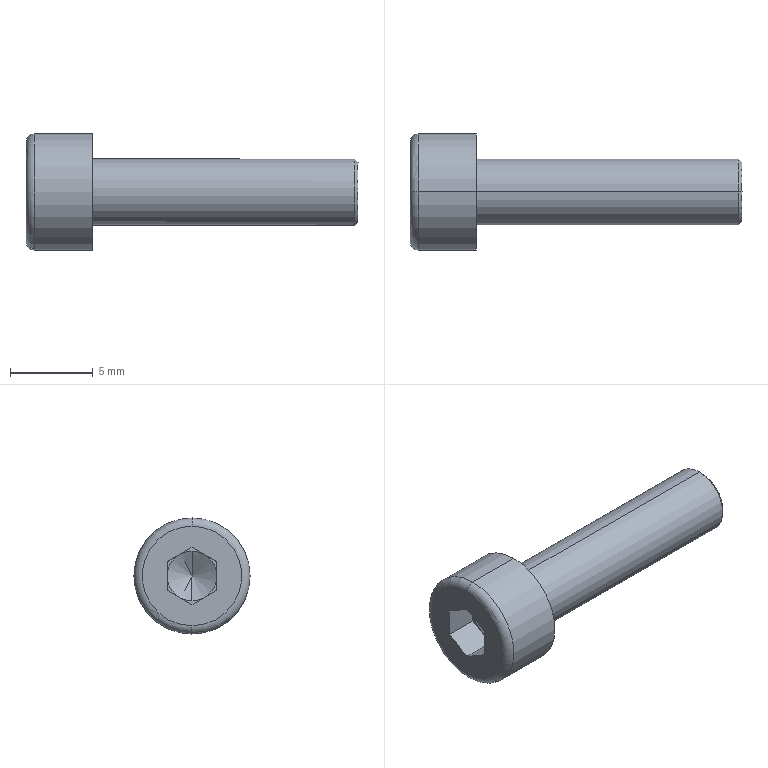Component | SolidWorks | hexagon socket head cap screws gb-34 | 1 solid | 25 faces | box 20.01 x 7 x 7 mm | volume 336 mm3 | plane 15 | cone 4 | cylinder 4 | torus 2 | commonest cylinder face diameters 4 x2 7 x2
STEP:
#1=CARTESIAN_POINT('',(-1.336,35.871,32.265));
#2=VERTEX_POINT('',#1);
#3=CARTESIAN_POINT('',(-1.336,35.871,32.407));
#4=VERTEX_POINT('',#3);
#5=CARTESIAN_POINT('',(-1.336,35.871,32.336));
#6=DIRECTION('',(1.,0.,-0.00108));
#7=DIRECTION('',(-0.00108,0.,-1.));
#8=AXIS2_PLACEMENT_3D('',#5,#6,#7);
#9=CIRCLE('',#8,0.07087);
#10=EDGE_CURVE('',#2,#4,#9,.T.);
#11=ORIENTED_EDGE('',*,*,#10,.F.);
#12=CARTESIAN_POINT('',(-1.344,35.871,32.257));
#13=VERTEX_POINT('',#12);
#14=CARTESIAN_POINT('',(-1.336,35.871,32.265));
#15=DIRECTION('',(-0.7079,0.,-0.7063));
#16=VECTOR('',#15,39.37);
#17=LINE('',#14,#16);
#18=EDGE_CURVE('',#2,#13,#17,.T.);
#19=ORIENTED_EDGE('',*,*,#18,.T.);
#20=CARTESIAN_POINT('',(-1.344,35.871,32.415));
#21=VERTEX_POINT('',#20);
#22=CARTESIAN_POINT('',(-1.344,35.871,32.336));
#23=DIRECTION('',(-1.,-0.,0.00108));
#24=DIRECTION('',(-0.00108,0.,-1.));
#25=AXIS2_PLACEMENT_3D('',#22,#23,#24);
#26=CIRCLE('',#25,0.07874);
#27=EDGE_CURVE('',#21,#13,#26,.T.);
#28=ORIENTED_EDGE('',*,*,#27,.F.);
#29=CARTESIAN_POINT('',(-1.336,35.871,32.407));
#30=DIRECTION('',(-0.7063,-0.,0.7079));
#31=VECTOR('',#30,39.37);
#32=LINE('',#29,#31);
#33=EDGE_CURVE('',#4,#21,#32,.T.);
#34=ORIENTED_EDGE('',*,*,#33,.F.);
#35=EDGE_LOOP('',(#11,#19,#28,#34));
#36=FACE_OUTER_BOUND('',#35,.T.);
#37=CARTESIAN_POINT('',(-1.336,35.871,32.336));
#38=DIRECTION('',(-1.,-0.,0.00108));
#39=DIRECTION('',(0.00108,-0.,1.));
#40=AXIS2_PLACEMENT_3D('',#37,#38,#39);
#41=CONICAL_SURFACE('',#40,0.07087,0.7854);
#42=ADVANCED_FACE('',(#36),#41,.T.);
#43=CARTESIAN_POINT('',(-2.123,35.871,32.455));
#44=VERTEX_POINT('',#43);
#45=CARTESIAN_POINT('',(-2.124,35.871,32.219));
#46=VERTEX_POINT('',#45);
#47=CARTESIAN_POINT('',(-2.123,35.871,32.337));
#48=DIRECTION('',(-1.,-0.,0.00108));
#49=DIRECTION('',(-0.00108,0.,-1.));
#50=AXIS2_PLACEMENT_3D('',#47,#48,#49);
#51=CIRCLE('',#50,0.1181);
#52=EDGE_CURVE('',#44,#46,#51,.T.);
#53=ORIENTED_EDGE('',*,*,#52,.F.);
#54=CARTESIAN_POINT('',(-2.104,35.871,32.475));
#55=VERTEX_POINT('',#54);
#56=CARTESIAN_POINT('',(-2.104,35.871,32.455));
#57=DIRECTION('',(0.,1.,0.));
#58=DIRECTION('',(0.,-0.,1.));
#59=AXIS2_PLACEMENT_3D('',#56,#57,#58);
#60=CIRCLE('',#59,0.01969);
#61=EDGE_CURVE('',#44,#55,#60,.T.);
#62=ORIENTED_EDGE('',*,*,#61,.T.);
#63=CARTESIAN_POINT('',(-2.104,35.871,32.199));
#64=VERTEX_POINT('',#63);
#65=CARTESIAN_POINT('',(-2.104,35.871,32.337));
#66=DIRECTION('',(1.,0.,-0.00108));
#67=DIRECTION('',(-0.00108,0.,-1.));
#68=AXIS2_PLACEMENT_3D('',#65,#66,#67);
#69=CIRCLE('',#68,0.1378);
#70=EDGE_CURVE('',#64,#55,#69,.T.);
#71=ORIENTED_EDGE('',*,*,#70,.F.);
#72=CARTESIAN_POINT('',(-2.104,35.871,32.219));
#73=DIRECTION('',(-0.,-1.,-0.));
#74=DIRECTION('',(0.,0.,-1.));
#75=AXIS2_PLACEMENT_3D('',#72,#73,#74);
#76=CIRCLE('',#75,0.01969);
#77=EDGE_CURVE('',#46,#64,#76,.T.);
#78=ORIENTED_EDGE('',*,*,#77,.F.);
#79=EDGE_LOOP('',(#53,#62,#71,#78));
#80=FACE_OUTER_BOUND('',#79,.T.);
#81=CARTESIAN_POINT('',(-2.104,35.871,32.337));
#82=DIRECTION('',(1.,0.,-0.00108));
#83=DIRECTION('',(-0.00108,0.,-1.));
#84=AXIS2_PLACEMENT_3D('',#81,#82,#83);
#85=TOROIDAL_SURFACE('',#84,0.1181,0.01969);
#86=ADVANCED_FACE('',(#80),#85,.T.);
#87=CARTESIAN_POINT('',(-2.011,35.871,32.337));
#88=VERTEX_POINT('',#87);
#89=CARTESIAN_POINT('',(-2.045,35.871,32.396));
#90=VERTEX_POINT('',#89);
#91=CARTESIAN_POINT('',(-2.045,35.871,32.396));
#92=DIRECTION('',(-0.4991,-0.,0.8666));
#93=VECTOR('',#92,39.37);
#94=LINE('',#91,#93);
#95=EDGE_CURVE('',#88,#90,#94,.T.);
#96=ORIENTED_EDGE('',*,*,#95,.F.);
#97=CARTESIAN_POINT('',(-2.045,35.871,32.278));
#98=VERTEX_POINT('',#97);
#99=CARTESIAN_POINT('',(-2.045,35.871,32.278));
#100=DIRECTION('',(-0.5009,0.,-0.8655));
#101=VECTOR('',#100,39.37);
#102=LINE('',#99,#101);
#103=EDGE_CURVE('',#88,#98,#102,.T.);
#104=ORIENTED_EDGE('',*,*,#103,.T.);
#105=CARTESIAN_POINT('',(-2.045,35.841,32.286));
#106=VERTEX_POINT('',#105);
#107=CARTESIAN_POINT('',(-2.045,35.871,32.337));
#108=DIRECTION('',(1.,0.,-0.00108));
#109=DIRECTION('',(0.00108,-0.,1.));
#110=AXIS2_PLACEMENT_3D('',#107,#108,#109);
#111=CIRCLE('',#110,0.05906);
#112=EDGE_CURVE('',#106,#98,#111,.T.);
#113=ORIENTED_EDGE('',*,*,#112,.F.);
#114=CARTESIAN_POINT('',(-2.045,35.811,32.337));
#115=VERTEX_POINT('',#114);
#116=CARTESIAN_POINT('',(-2.045,35.871,32.337));
#117=DIRECTION('',(1.,0.,-0.00108));
#118=DIRECTION('',(0.00108,-0.,1.));
#119=AXIS2_PLACEMENT_3D('',#116,#117,#118);
#120=CIRCLE('',#119,0.05906);
#121=EDGE_CURVE('',#115,#106,#120,.T.);
#122=ORIENTED_EDGE('',*,*,#121,.F.);
#123=CARTESIAN_POINT('',(-2.045,35.841,32.388));
#124=VERTEX_POINT('',#123);
#125=CARTESIAN_POINT('',(-2.045,35.871,32.337));
#126=DIRECTION('',(1.,0.,-0.00108));
#127=DIRECTION('',(0.00108,-0.,1.));
#128=AXIS2_PLACEMENT_3D('',#125,#126,#127);
#129=CIRCLE('',#128,0.05906);
#130=EDGE_CURVE('',#124,#115,#129,.T.);
#131=ORIENTED_EDGE('',*,*,#130,.F.);
#132=CARTESIAN_POINT('',(-2.045,35.871,32.337));
#133=DIRECTION('',(1.,0.,-0.00108));
#134=DIRECTION('',(0.00108,-0.,1.));
#135=AXIS2_PLACEMENT_3D('',#132,#133,#134);
#136=CIRCLE('',#135,0.05906);
#137=EDGE_CURVE('',#90,#124,#136,.T.);
#138=ORIENTED_EDGE('',*,*,#137,.F.);
#139=EDGE_LOOP('',(#96,#104,#113,#122,#131,#138));
#140=FACE_OUTER_BOUND('',#139,.T.);
#141=CARTESIAN_POINT('',(-2.045,35.871,32.337));
#142=DIRECTION('',(-1.,-0.,0.00108));
#143=DIRECTION('',(0.00108,-0.,1.));
#144=AXIS2_PLACEMENT_3D('',#141,#142,#143);
#145=CONICAL_SURFACE('',#144,0.05906,1.047);
#146=ADVANCED_FACE('',(#140),#145,.F.);
#147=ORIENTED_EDGE('',*,*,#27,.T.);
#148=CARTESIAN_POINT('',(-1.966,35.871,32.258));
#149=VERTEX_POINT('',#148);
#150=CARTESIAN_POINT('',(-1.336,35.871,32.257));
#151=DIRECTION('',(-1.,-0.,0.00108));
#152=VECTOR('',#151,39.37);
#153=LINE('',#150,#152);
#154=EDGE_CURVE('',#13,#149,#153,.T.);
#155=ORIENTED_EDGE('',*,*,#154,.T.);
#156=CARTESIAN_POINT('',(-1.966,35.871,32.415));
#157=VERTEX_POINT('',#156);
#158=CARTESIAN_POINT('',(-1.966,35.871,32.337));
#159=DIRECTION('',(1.,0.,-0.00108));
#160=DIRECTION('',(-0.00108,0.,-1.));
#161=AXIS2_PLACEMENT_3D('',#158,#159,#160);
#162=CIRCLE('',#161,0.07874);
#163=EDGE_CURVE('',#149,#157,#162,.T.);
#164=ORIENTED_EDGE('',*,*,#163,.T.);
#165=CARTESIAN_POINT('',(-1.336,35.871,32.415));
#166=DIRECTION('',(-1.,-0.,0.00108));
#167=VECTOR('',#166,39.37);
#168=LINE('',#165,#167);
#169=EDGE_CURVE('',#21,#157,#168,.T.);
#170=ORIENTED_EDGE('',*,*,#169,.F.);
#171=EDGE_LOOP('',(#147,#155,#164,#170));
#172=FACE_OUTER_BOUND('',#171,.T.);
#173=CARTESIAN_POINT('',(-1.336,35.871,32.336));
#174=DIRECTION('',(-1.,-0.,0.00108));
#175=DIRECTION('',(0.00108,-0.,1.));
#176=AXIS2_PLACEMENT_3D('',#173,#174,#175);
#177=CYLINDRICAL_SURFACE('',#176,0.07874);
#178=ADVANCED_FACE('',(#172),#177,.T.);
#179=CARTESIAN_POINT('',(-1.966,35.871,32.199));
#180=VERTEX_POINT('',#179);
#181=CARTESIAN_POINT('',(-1.966,35.871,32.474));
#182=VERTEX_POINT('',#181);
#183=CARTESIAN_POINT('',(-1.966,35.871,32.337));
#184=DIRECTION('',(1.,0.,-0.00108));
#185=DIRECTION('',(-0.00108,0.,-1.));
#186=AXIS2_PLACEMENT_3D('',#183,#184,#185);
#187=CIRCLE('',#186,0.1378);
#188=EDGE_CURVE('',#180,#182,#187,.T.);
#189=ORIENTED_EDGE('',*,*,#188,.F.);
#190=CARTESIAN_POINT('',(-1.966,35.871,32.199));
#191=DIRECTION('',(-1.,-0.,0.00108));
#192=VECTOR('',#191,39.37);
#193=LINE('',#190,#192);
#194=EDGE_CURVE('',#180,#64,#193,.T.);
#195=ORIENTED_EDGE('',*,*,#194,.T.);
#196=ORIENTED_EDGE('',*,*,#70,.T.);
#197=CARTESIAN_POINT('',(-1.966,35.871,32.474));
#198=DIRECTION('',(-1.,-0.,0.00108));
#199=VECTOR('',#198,39.37);
#200=LINE('',#197,#199);
#201=EDGE_CURVE('',#182,#55,#200,.T.);
#202=ORIENTED_EDGE('',*,*,#201,.F.);
#203=EDGE_LOOP('',(#189,#195,#196,#202));
#204=FACE_OUTER_BOUND('',#203,.T.);
#205=CARTESIAN_POINT('',(-1.966,35.871,32.337));
#206=DIRECTION('',(-1.,-0.,0.00108));
#207=DIRECTION('',(0.00108,-0.,1.));
#208=AXIS2_PLACEMENT_3D('',#205,#206,#207);
#209=CYLINDRICAL_SURFACE('',#208,0.1378);
#210=ADVANCED_FACE('',(#204),#209,.T.);
#211=CARTESIAN_POINT('',(-2.045,35.811,32.371));
#212=VERTEX_POINT('',#211);
#213=CARTESIAN_POINT('',(-2.045,35.871,32.405));
#214=DIRECTION('',(-0.0005402,-0.866,-0.5));
#215=VECTOR('',#214,39.37);
#216=LINE('',#213,#215);
#217=EDGE_CURVE('',#124,#212,#216,.T.);
#218=ORIENTED_EDGE('',*,*,#217,.F.);
#219=ORIENTED_EDGE('',*,*,#130,.T.);
#220=CARTESIAN_POINT('',(-2.045,35.811,32.371));
#221=DIRECTION('',(-0.00108,0.,-1.));
#222=VECTOR('',#221,39.37);
#223=LINE('',#220,#222);
#224=EDGE_CURVE('',#212,#115,#223,.T.);
#225=ORIENTED_EDGE('',*,*,#224,.F.);
#226=EDGE_LOOP('',(#218,#219,#225));
#227=FACE_OUTER_BOUND('',#226,.T.);
#228=CARTESIAN_POINT('',(-2.045,35.752,32.337));
#229=DIRECTION('',(-1.,-0.,0.00108));
#230=DIRECTION('',(0.00108,-0.,1.));
#231=AXIS2_PLACEMENT_3D('',#228,#229,#230);
#232=PLANE('',#231);
#233=ADVANCED_FACE('',(#227),#232,.T.);
#234=CARTESIAN_POINT('',(-2.045,35.811,32.303));
#235=VERTEX_POINT('',#234);
#236=CARTESIAN_POINT('',(-2.045,35.811,32.371));
#237=DIRECTION('',(-0.00108,0.,-1.));
#238=VECTOR('',#237,39.37);
#239=LINE('',#236,#238);
#240=EDGE_CURVE('',#115,#235,#239,.T.);
#241=ORIENTED_EDGE('',*,*,#240,.F.);
#242=ORIENTED_EDGE('',*,*,#121,.T.);
#243=CARTESIAN_POINT('',(-2.045,35.811,32.303));
#244=DIRECTION('',(-0.0005402,0.866,-0.5));
#245=VECTOR('',#244,39.37);
#246=LINE('',#243,#245);
#247=EDGE_CURVE('',#235,#106,#246,.T.);
#248=ORIENTED_EDGE('',*,*,#247,.F.);
#249=EDGE_LOOP('',(#241,#242,#248));
#250=FACE_OUTER_BOUND('',#249,.T.);
#251=CARTESIAN_POINT('',(-2.045,35.752,32.337));
#252=DIRECTION('',(-1.,-0.,0.00108));
#253=DIRECTION('',(0.00108,-0.,1.));
#254=AXIS2_PLACEMENT_3D('',#251,#252,#253);
#255=PLANE('',#254);
#256=ADVANCED_FACE('',(#250),#255,.T.);
#257=CARTESIAN_POINT('',(-2.045,35.871,32.269));
#258=VERTEX_POINT('',#257);
#259=CARTESIAN_POINT('',(-2.045,35.811,32.303));
#260=DIRECTION('',(-0.0005402,0.866,-0.5));
#261=VECTOR('',#260,39.37);
#262=LINE('',#259,#261);
#263=EDGE_CURVE('',#106,#258,#262,.T.);
#264=ORIENTED_EDGE('',*,*,#263,.F.);
#265=ORIENTED_EDGE('',*,*,#112,.T.);
#266=CARTESIAN_POINT('',(-2.045,35.9,32.286));
#267=VERTEX_POINT('',#266);
#268=CARTESIAN_POINT('',(-2.045,35.871,32.337));
#269=DIRECTION('',(1.,0.,-0.00108));
#270=DIRECTION('',(0.00108,-0.,1.));
#271=AXIS2_PLACEMENT_3D('',#268,#269,#270);
#272=CIRCLE('',#271,0.05906);
#273=EDGE_CURVE('',#98,#267,#272,.T.);
#274=ORIENTED_EDGE('',*,*,#273,.T.);
#275=CARTESIAN_POINT('',(-2.045,35.871,32.269));
#276=DIRECTION('',(0.0005402,0.866,0.5));
#277=VECTOR('',#276,39.37);
#278=LINE('',#275,#277);
#279=EDGE_CURVE('',#258,#267,#278,.T.);
#280=ORIENTED_EDGE('',*,*,#279,.F.);
#281=EDGE_LOOP('',(#264,#265,#274,#280));
#282=FACE_OUTER_BOUND('',#281,.T.);
#283=CARTESIAN_POINT('',(-2.045,35.752,32.337));
#284=DIRECTION('',(-1.,-0.,0.00108));
#285=DIRECTION('',(0.00108,-0.,1.));
#286=AXIS2_PLACEMENT_3D('',#283,#284,#285);
#287=PLANE('',#286);
#288=ADVANCED_FACE('',(#282),#287,.T.);
#289=CARTESIAN_POINT('',(-2.045,35.93,32.303));
#290=VERTEX_POINT('',#289);
#291=CARTESIAN_POINT('',(-2.045,35.871,32.269));
#292=DIRECTION('',(0.0005402,0.866,0.5));
#293=VECTOR('',#292,39.37);
#294=LINE('',#291,#293);
#295=EDGE_CURVE('',#267,#290,#294,.T.);
#296=ORIENTED_EDGE('',*,*,#295,.F.);
#297=CARTESIAN_POINT('',(-2.045,35.93,32.337));
#298=VERTEX_POINT('',#297);
#299=CARTESIAN_POINT('',(-2.045,35.871,32.337));
#300=DIRECTION('',(1.,0.,-0.00108));
#301=DIRECTION('',(-0.00108,0.,-1.));
#302=AXIS2_PLACEMENT_3D('',#299,#300,#301);
#303=CIRCLE('',#302,0.05906);
#304=EDGE_CURVE('',#267,#298,#303,.T.);
#305=ORIENTED_EDGE('',*,*,#304,.T.);
#306=CARTESIAN_POINT('',(-2.045,35.93,32.303));
#307=DIRECTION('',(0.00108,-0.,1.));
#308=VECTOR('',#307,39.37);
#309=LINE('',#306,#308);
#310=EDGE_CURVE('',#290,#298,#309,.T.);
#311=ORIENTED_EDGE('',*,*,#310,.F.);
#312=EDGE_LOOP('',(#296,#305,#311));
#313=FACE_OUTER_BOUND('',#312,.T.);
#314=CARTESIAN_POINT('',(-2.045,35.752,32.337));
#315=DIRECTION('',(-1.,-0.,0.00108));
#316=DIRECTION('',(0.00108,-0.,1.));
#317=AXIS2_PLACEMENT_3D('',#314,#315,#316);
#318=PLANE('',#317);
#319=ADVANCED_FACE('',(#313),#318,.T.);
#320=CARTESIAN_POINT('',(-2.045,35.93,32.371));
#321=VERTEX_POINT('',#320);
#322=CARTESIAN_POINT('',(-2.045,35.93,32.303));
#323=DIRECTION('',(0.00108,-0.,1.));
#324=VECTOR('',#323,39.37);
#325=LINE('',#322,#324);
#326=EDGE_CURVE('',#298,#321,#325,.T.);
#327=ORIENTED_EDGE('',*,*,#326,.F.);
#328=CARTESIAN_POINT('',(-2.045,35.9,32.388));
#329=VERTEX_POINT('',#328);
#330=CARTESIAN_POINT('',(-2.045,35.871,32.337));
#331=DIRECTION('',(1.,0.,-0.00108));
#332=DIRECTION('',(0.00108,-0.,1.));
#333=AXIS2_PLACEMENT_3D('',#330,#331,#332);
#334=CIRCLE('',#333,0.05906);
#335=EDGE_CURVE('',#298,#329,#334,.T.);
#336=ORIENTED_EDGE('',*,*,#335,.T.);
#337=CARTESIAN_POINT('',(-2.045,35.93,32.371));
#338=DIRECTION('',(0.0005402,-0.866,0.5));
#339=VECTOR('',#338,39.37);
#340=LINE('',#337,#339);
#341=EDGE_CURVE('',#321,#329,#340,.T.);
#342=ORIENTED_EDGE('',*,*,#341,.F.);
#343=EDGE_LOOP('',(#327,#336,#342));
#344=FACE_OUTER_BOUND('',#343,.T.);
#345=CARTESIAN_POINT('',(-2.045,35.752,32.337));
#346=DIRECTION('',(-1.,-0.,0.00108));
#347=DIRECTION('',(0.00108,-0.,1.));
#348=AXIS2_PLACEMENT_3D('',#345,#346,#347);
#349=PLANE('',#348);
#350=ADVANCED_FACE('',(#344),#349,.T.);
#351=CARTESIAN_POINT('',(-2.045,35.871,32.405));
#352=VERTEX_POINT('',#351);
#353=CARTESIAN_POINT('',(-2.045,35.93,32.371));
#354=DIRECTION('',(0.0005402,-0.866,0.5));
#355=VECTOR('',#354,39.37);
#356=LINE('',#353,#355);
#357=EDGE_CURVE('',#329,#352,#356,.T.);
#358=ORIENTED_EDGE('',*,*,#357,.F.);
#359=CARTESIAN_POINT('',(-2.045,35.871,32.337));
#360=DIRECTION('',(1.,0.,-0.00108));
#361=DIRECTION('',(0.00108,-0.,1.));
#362=AXIS2_PLACEMENT_3D('',#359,#360,#361);
#363=CIRCLE('',#362,0.05906);
#364=EDGE_CURVE('',#329,#90,#363,.T.);
#365=ORIENTED_EDGE('',*,*,#364,.T.);
#366=ORIENTED_EDGE('',*,*,#137,.T.);
#367=CARTESIAN_POINT('',(-2.045,35.871,32.405));
#368=DIRECTION('',(-0.0005402,-0.866,-0.5));
#369=VECTOR('',#368,39.37);
#370=LINE('',#367,#369);
#371=EDGE_CURVE('',#352,#124,#370,.T.);
#372=ORIENTED_EDGE('',*,*,#371,.F.);
#373=EDGE_LOOP('',(#358,#365,#366,#372));
#374=FACE_OUTER_BOUND('',#373,.T.);
#375=CARTESIAN_POINT('',(-2.045,35.752,32.337));
#376=DIRECTION('',(-1.,-0.,0.00108));
#377=DIRECTION('',(0.00108,-0.,1.));
#378=AXIS2_PLACEMENT_3D('',#375,#376,#377);
#379=PLANE('',#378);
#380=ADVANCED_FACE('',(#374),#379,.T.);
#381=CARTESIAN_POINT('',(-2.123,35.871,32.337));
#382=DIRECTION('',(-1.,-0.,0.00108));
#383=DIRECTION('',(-0.00108,0.,-1.));
#384=AXIS2_PLACEMENT_3D('',#381,#382,#383);
#385=CIRCLE('',#384,0.1181);
#386=EDGE_CURVE('',#46,#44,#385,.T.);
#387=ORIENTED_EDGE('',*,*,#386,.T.);
#388=ORIENTED_EDGE('',*,*,#52,.T.);
#389=EDGE_LOOP('',(#387,#388));
#390=FACE_OUTER_BOUND('',#389,.T.);
#391=CARTESIAN_POINT('',(-2.123,35.811,32.303));
#392=VERTEX_POINT('',#391);
#393=CARTESIAN_POINT('',(-2.123,35.871,32.269));
#394=VERTEX_POINT('',#393);
#395=CARTESIAN_POINT('',(-2.123,35.811,32.303));
#396=DIRECTION('',(-0.0005402,0.866,-0.5));
#397=VECTOR('',#396,39.37);
#398=LINE('',#395,#397);
#399=EDGE_CURVE('',#392,#394,#398,.T.);
#400=ORIENTED_EDGE('',*,*,#399,.T.);
#401=CARTESIAN_POINT('',(-2.123,35.93,32.303));
#402=VERTEX_POINT('',#401);
#403=CARTESIAN_POINT('',(-2.123,35.871,32.269));
#404=DIRECTION('',(0.0005402,0.866,0.5));
#405=VECTOR('',#404,39.37);
#406=LINE('',#403,#405);
#407=EDGE_CURVE('',#394,#402,#406,.T.);
#408=ORIENTED_EDGE('',*,*,#407,.T.);
#409=CARTESIAN_POINT('',(-2.123,35.93,32.371));
#410=VERTEX_POINT('',#409);
#411=CARTESIAN_POINT('',(-2.123,35.93,32.303));
#412=DIRECTION('',(0.00108,-0.,1.));
#413=VECTOR('',#412,39.37);
#414=LINE('',#411,#413);
#415=EDGE_CURVE('',#402,#410,#414,.T.);
#416=ORIENTED_EDGE('',*,*,#415,.T.);
#417=CARTESIAN_POINT('',(-2.123,35.871,32.405));
#418=VERTEX_POINT('',#417);
#419=CARTESIAN_POINT('',(-2.123,35.93,32.371));
#420=DIRECTION('',(0.0005402,-0.866,0.5));
#421=VECTOR('',#420,39.37);
#422=LINE('',#419,#421);
#423=EDGE_CURVE('',#410,#418,#422,.T.);
#424=ORIENTED_EDGE('',*,*,#423,.T.);
#425=CARTESIAN_POINT('',(-2.123,35.811,32.371));
#426=VERTEX_POINT('',#425);
#427=CARTESIAN_POINT('',(-2.123,35.871,32.405));
#428=DIRECTION('',(-0.0005402,-0.866,-0.5));
#429=VECTOR('',#428,39.37);
#430=LINE('',#427,#429);
#431=EDGE_CURVE('',#418,#426,#430,.T.);
#432=ORIENTED_EDGE('',*,*,#431,.T.);
#433=CARTESIAN_POINT('',(-2.123,35.811,32.371));
#434=DIRECTION('',(-0.00108,0.,-1.));
#435=VECTOR('',#434,39.37);
#436=LINE('',#433,#435);
#437=EDGE_CURVE('',#426,#392,#436,.T.);
#438=ORIENTED_EDGE('',*,*,#437,.T.);
#439=EDGE_LOOP('',(#400,#408,#416,#424,#432,#438));
#440=FACE_BOUND('',#439,.T.);
#441=CARTESIAN_POINT('',(-2.123,35.871,32.337));
#442=DIRECTION('',(1.,0.,-0.00108));
#443=DIRECTION('',(-0.00108,0.,-1.));
#444=AXIS2_PLACEMENT_3D('',#441,#442,#443);
#445=PLANE('',#444);
#446=ADVANCED_FACE('',(#390,#440),#445,.F.);
#447=CARTESIAN_POINT('',(-1.966,35.871,32.337));
#448=DIRECTION('',(1.,0.,-0.00108));
#449=DIRECTION('',(-0.00108,0.,-1.));
#450=AXIS2_PLACEMENT_3D('',#447,#448,#449);
#451=CIRCLE('',#450,0.1378);
#452=EDGE_CURVE('',#182,#180,#451,.T.);
#453=ORIENTED_EDGE('',*,*,#452,.T.);
#454=ORIENTED_EDGE('',*,*,#188,.T.);
#455=EDGE_LOOP('',(#453,#454));
#456=FACE_OUTER_BOUND('',#455,.T.);
#457=CARTESIAN_POINT('',(-1.966,35.871,32.337));
#458=DIRECTION('',(1.,0.,-0.00108));
#459=DIRECTION('',(-0.00108,0.,-1.));
#460=AXIS2_PLACEMENT_3D('',#457,#458,#459);
#461=CIRCLE('',#460,0.07874);
#462=EDGE_CURVE('',#157,#149,#461,.T.);
#463=ORIENTED_EDGE('',*,*,#462,.F.);
#464=ORIENTED_EDGE('',*,*,#163,.F.);
#465=EDGE_LOOP('',(#463,#464));
#466=FACE_BOUND('',#465,.T.);
#467=CARTESIAN_POINT('',(-1.966,35.871,32.337));
#468=DIRECTION('',(1.,0.,-0.00108));
#469=DIRECTION('',(-0.00108,0.,-1.));
#470=AXIS2_PLACEMENT_3D('',#467,#468,#469);
#471=PLANE('',#470);
#472=ADVANCED_FACE('',(#456,#466),#471,.T.);
#473=ORIENTED_EDGE('',*,*,#194,.F.);
#474=ORIENTED_EDGE('',*,*,#452,.F.);
#475=ORIENTED_EDGE('',*,*,#201,.T.);
#476=CARTESIAN_POINT('',(-2.104,35.871,32.337));
#477=DIRECTION('',(1.,0.,-0.00108));
#478=DIRECTION('',(-0.00108,0.,-1.));
#479=AXIS2_PLACEMENT_3D('',#476,#477,#478);
#480=CIRCLE('',#479,0.1378);
#481=EDGE_CURVE('',#55,#64,#480,.T.);
#482=ORIENTED_EDGE('',*,*,#481,.T.);
#483=EDGE_LOOP('',(#473,#474,#475,#482));
#484=FACE_OUTER_BOUND('',#483,.T.);
#485=CARTESIAN_POINT('',(-1.966,35.871,32.337));
#486=DIRECTION('',(-1.,-0.,0.00108));
#487=DIRECTION('',(0.00108,-0.,1.));
#488=AXIS2_PLACEMENT_3D('',#485,#486,#487);
#489=CYLINDRICAL_SURFACE('',#488,0.1378);
#490=ADVANCED_FACE('',(#484),#489,.T.);
#491=ORIENTED_EDGE('',*,*,#154,.F.);
#492=CARTESIAN_POINT('',(-1.344,35.871,32.336));
#493=DIRECTION('',(-1.,-0.,0.00108));
#494=DIRECTION('',(-0.00108,0.,-1.));
#495=AXIS2_PLACEMENT_3D('',#492,#493,#494);
#496=CIRCLE('',#495,0.07874);
#497=EDGE_CURVE('',#13,#21,#496,.T.);
#498=ORIENTED_EDGE('',*,*,#497,.T.);
#499=ORIENTED_EDGE('',*,*,#169,.T.);
#500=ORIENTED_EDGE('',*,*,#462,.T.);
#501=EDGE_LOOP('',(#491,#498,#499,#500));
#502=FACE_OUTER_BOUND('',#501,.T.);
#503=CARTESIAN_POINT('',(-1.336,35.871,32.336));
#504=DIRECTION('',(-1.,-0.,0.00108));
#505=DIRECTION('',(0.00108,-0.,1.));
#506=AXIS2_PLACEMENT_3D('',#503,#504,#505);
#507=CYLINDRICAL_SURFACE('',#506,0.07874);
#508=ADVANCED_FACE('',(#502),#507,.T.);
#509=CARTESIAN_POINT('',(-1.336,35.871,32.336));
#510=DIRECTION('',(1.,0.,-0.00108));
#511=DIRECTION('',(-0.00108,0.,-1.));
#512=AXIS2_PLACEMENT_3D('',#509,#510,#511);
#513=CIRCLE('',#512,0.07087);
#514=EDGE_CURVE('',#4,#2,#513,.T.);
#515=ORIENTED_EDGE('',*,*,#514,.T.);
#516=ORIENTED_EDGE('',*,*,#10,.T.);
#517=EDGE_LOOP('',(#515,#516));
#518=FACE_OUTER_BOUND('',#517,.T.);
#519=CARTESIAN_POINT('',(-1.336,35.871,32.336));
#520=DIRECTION('',(1.,0.,-0.00108));
#521=DIRECTION('',(-0.00108,0.,-1.));
#522=AXIS2_PLACEMENT_3D('',#519,#520,#521);
#523=PLANE('',#522);
#524=ADVANCED_FACE('',(#518),#523,.T.);
#525=ORIENTED_EDGE('',*,*,#399,.F.);
#526=CARTESIAN_POINT('',(-2.045,35.811,32.303));
#527=DIRECTION('',(-1.,-0.,0.00108));
#528=VECTOR('',#527,39.37);
#529=LINE('',#526,#528);
#530=EDGE_CURVE('',#235,#392,#529,.T.);
#531=ORIENTED_EDGE('',*,*,#530,.F.);
#532=ORIENTED_EDGE('',*,*,#247,.T.);
#533=ORIENTED_EDGE('',*,*,#263,.T.);
#534=CARTESIAN_POINT('',(-2.045,35.871,32.269));
#535=DIRECTION('',(-1.,-0.,0.00108));
#536=VECTOR('',#535,39.37);
#537=LINE('',#534,#536);
#538=EDGE_CURVE('',#258,#394,#537,.T.);
#539=ORIENTED_EDGE('',*,*,#538,.T.);
#540=EDGE_LOOP('',(#525,#531,#532,#533,#539));
#541=FACE_OUTER_BOUND('',#540,.T.);
#542=CARTESIAN_POINT('',(-2.045,35.811,32.303));
#543=DIRECTION('',(0.0009357,0.5,0.866));
#544=DIRECTION('',(0.0005402,-0.866,0.5));
#545=AXIS2_PLACEMENT_3D('',#542,#543,#544);
#546=PLANE('',#545);
#547=ADVANCED_FACE('',(#541),#546,.T.);
#548=ORIENTED_EDGE('',*,*,#407,.F.);
#549=ORIENTED_EDGE('',*,*,#538,.F.);
#550=ORIENTED_EDGE('',*,*,#279,.T.);
#551=ORIENTED_EDGE('',*,*,#295,.T.);
#552=CARTESIAN_POINT('',(-2.045,35.93,32.303));
#553=DIRECTION('',(-1.,-0.,0.00108));
#554=VECTOR('',#553,39.37);
#555=LINE('',#552,#554);
#556=EDGE_CURVE('',#290,#402,#555,.T.);
#557=ORIENTED_EDGE('',*,*,#556,.T.);
#558=EDGE_LOOP('',(#548,#549,#550,#551,#557));
#559=FACE_OUTER_BOUND('',#558,.T.);
#560=CARTESIAN_POINT('',(-2.045,35.871,32.269));
#561=DIRECTION('',(0.0009357,-0.5,0.866));
#562=DIRECTION('',(-0.0005402,-0.866,-0.5));
#563=AXIS2_PLACEMENT_3D('',#560,#561,#562);
#564=PLANE('',#563);
#565=ADVANCED_FACE('',(#559),#564,.T.);
#566=ORIENTED_EDGE('',*,*,#415,.F.);
#567=ORIENTED_EDGE('',*,*,#556,.F.);
#568=ORIENTED_EDGE('',*,*,#310,.T.);
#569=ORIENTED_EDGE('',*,*,#326,.T.);
#570=CARTESIAN_POINT('',(-2.045,35.93,32.371));
#571=DIRECTION('',(-1.,-0.,0.00108));
#572=VECTOR('',#571,39.37);
#573=LINE('',#570,#572);
#574=EDGE_CURVE('',#321,#410,#573,.T.);
#575=ORIENTED_EDGE('',*,*,#574,.T.);
#576=EDGE_LOOP('',(#566,#567,#568,#569,#575));
#577=FACE_OUTER_BOUND('',#576,.T.);
#578=CARTESIAN_POINT('',(-2.045,35.93,32.303));
#579=DIRECTION('',(-0.,-1.,-0.));
#580=DIRECTION('',(-0.00108,0.,-1.));
#581=AXIS2_PLACEMENT_3D('',#578,#579,#580);
#582=PLANE('',#581);
#583=ADVANCED_FACE('',(#577),#582,.T.);
#584=ORIENTED_EDGE('',*,*,#423,.F.);
#585=ORIENTED_EDGE('',*,*,#574,.F.);
#586=ORIENTED_EDGE('',*,*,#341,.T.);
#587=ORIENTED_EDGE('',*,*,#357,.T.);
#588=CARTESIAN_POINT('',(-2.045,35.871,32.405));
#589=DIRECTION('',(-1.,-0.,0.00108));
#590=VECTOR('',#589,39.37);
#591=LINE('',#588,#590);
#592=EDGE_CURVE('',#352,#418,#591,.T.);
#593=ORIENTED_EDGE('',*,*,#592,.T.);
#594=EDGE_LOOP('',(#584,#585,#586,#587,#593));
#595=FACE_OUTER_BOUND('',#594,.T.);
#596=CARTESIAN_POINT('',(-2.045,35.93,32.371));
#597=DIRECTION('',(-0.0009357,-0.5,-0.866));
#598=DIRECTION('',(-0.0005402,0.866,-0.5));
#599=AXIS2_PLACEMENT_3D('',#596,#597,#598);
#600=PLANE('',#599);
#601=ADVANCED_FACE('',(#595),#600,.T.);
#602=ORIENTED_EDGE('',*,*,#431,.F.);
#603=ORIENTED_EDGE('',*,*,#592,.F.);
#604=ORIENTED_EDGE('',*,*,#371,.T.);
#605=ORIENTED_EDGE('',*,*,#217,.T.);
#606=CARTESIAN_POINT('',(-2.045,35.811,32.371));
#607=DIRECTION('',(-1.,-0.,0.00108));
#608=VECTOR('',#607,39.37);
#609=LINE('',#606,#608);
#610=EDGE_CURVE('',#212,#426,#609,.T.);
#611=ORIENTED_EDGE('',*,*,#610,.T.);
#612=EDGE_LOOP('',(#602,#603,#604,#605,#611));
#613=FACE_OUTER_BOUND('',#612,.T.);
#614=CARTESIAN_POINT('',(-2.045,35.871,32.405));
#615=DIRECTION('',(-0.0009357,0.5,-0.866));
#616=DIRECTION('',(0.0005402,0.866,0.5));
#617=AXIS2_PLACEMENT_3D('',#614,#615,#616);
#618=PLANE('',#617);
#619=ADVANCED_FACE('',(#613),#618,.T.);
#620=ORIENTED_EDGE('',*,*,#437,.F.);
#621=ORIENTED_EDGE('',*,*,#610,.F.);
#622=ORIENTED_EDGE('',*,*,#224,.T.);
#623=ORIENTED_EDGE('',*,*,#240,.T.);
#624=ORIENTED_EDGE('',*,*,#530,.T.);
#625=EDGE_LOOP('',(#620,#621,#622,#623,#624));
#626=FACE_OUTER_BOUND('',#625,.T.);
#627=CARTESIAN_POINT('',(-2.045,35.811,32.371));
#628=DIRECTION('',(0.,1.,0.));
#629=DIRECTION('',(0.00108,-0.,1.));
#630=AXIS2_PLACEMENT_3D('',#627,#628,#629);
#631=PLANE('',#630);
#632=ADVANCED_FACE('',(#626),#631,.T.);
#633=ORIENTED_EDGE('',*,*,#103,.F.);
#634=ORIENTED_EDGE('',*,*,#95,.T.);
#635=ORIENTED_EDGE('',*,*,#364,.F.);
#636=ORIENTED_EDGE('',*,*,#335,.F.);
#637=ORIENTED_EDGE('',*,*,#304,.F.);
#638=ORIENTED_EDGE('',*,*,#273,.F.);
#639=EDGE_LOOP('',(#633,#634,#635,#636,#637,#638));
#640=FACE_OUTER_BOUND('',#639,.T.);
#641=CARTESIAN_POINT('',(-2.045,35.871,32.337));
#642=DIRECTION('',(-1.,-0.,0.00108));
#643=DIRECTION('',(0.00108,-0.,1.));
#644=AXIS2_PLACEMENT_3D('',#641,#642,#643);
#645=CONICAL_SURFACE('',#644,0.05906,1.047);
#646=ADVANCED_FACE('',(#640),#645,.F.);
#647=ORIENTED_EDGE('',*,*,#61,.F.);
#648=ORIENTED_EDGE('',*,*,#386,.F.);
#649=ORIENTED_EDGE('',*,*,#77,.T.);
#650=ORIENTED_EDGE('',*,*,#481,.F.);
#651=EDGE_LOOP('',(#647,#648,#649,#650));
#652=FACE_OUTER_BOUND('',#651,.T.);
#653=CARTESIAN_POINT('',(-2.104,35.871,32.337));
#654=DIRECTION('',(1.,0.,-0.00108));
#655=DIRECTION('',(-0.00108,0.,-1.));
#656=AXIS2_PLACEMENT_3D('',#653,#654,#655);
#657=TOROIDAL_SURFACE('',#656,0.1181,0.01969);
#658=ADVANCED_FACE('',(#652),#657,.T.);
#659=ORIENTED_EDGE('',*,*,#18,.F.);
#660=ORIENTED_EDGE('',*,*,#514,.F.);
#661=ORIENTED_EDGE('',*,*,#33,.T.);
#662=ORIENTED_EDGE('',*,*,#497,.F.);
#663=EDGE_LOOP('',(#659,#660,#661,#662));
#664=FACE_OUTER_BOUND('',#663,.T.);
#665=CARTESIAN_POINT('',(-1.336,35.871,32.336));
#666=DIRECTION('',(-1.,-0.,0.00108));
#667=DIRECTION('',(0.00108,-0.,1.));
#668=AXIS2_PLACEMENT_3D('',#665,#666,#667);
#669=CONICAL_SURFACE('',#668,0.07087,0.7854);
#670=ADVANCED_FACE('',(#664),#669,.T.);
#671=CLOSED_SHELL('',(#42,#86,#146,#178,#210,#233,#256,#288,#319,#350,#380,#446,#472,#490,#508,#524,#547,#565,#583,#601,#619,#632,#646,#658,#670));
#672=MANIFOLD_SOLID_BREP('',#671);
#673=CARTESIAN_POINT('',(0.,0.,0.));
#674=DIRECTION('',(0.,0.,1.));
#675=DIRECTION('',(1.,0.,0.));
#676=AXIS2_PLACEMENT_3D('',#673,#674,#675);
#677=(LENGTH_UNIT()NAMED_UNIT(*)SI_UNIT($,.METRE.));
#678=LENGTH_MEASURE_WITH_UNIT(LENGTH_MEASURE(0.0254),#677);
#679=DIMENSIONAL_EXPONENTS(1.,0.,0.,0.,0.,0.,0.);
#680=(CONVERSION_BASED_UNIT('',#678)LENGTH_UNIT()NAMED_UNIT(#679));
#681=UNCERTAINTY_MEASURE_WITH_UNIT(LENGTH_MEASURE(0.00001),#680,'','');
#682=(NAMED_UNIT(*)PLANE_ANGLE_UNIT()SI_UNIT($,.RADIAN.));
#683=(NAMED_UNIT(*)SI_UNIT($,.STERADIAN.)SOLID_ANGLE_UNIT());
#684=(GEOMETRIC_REPRESENTATION_CONTEXT(3)GLOBAL_UNCERTAINTY_ASSIGNED_CONTEXT((#681))GLOBAL_UNIT_ASSIGNED_CONTEXT((#680,#682,#683))REPRESENTATION_CONTEXT('',''));
#685=ADVANCED_BREP_SHAPE_REPRESENTATION('',(#672,#676),#684);
#686=COLOUR_RGB('',0.7922,0.8196,0.9333);
#687=FILL_AREA_STYLE_COLOUR('',#686);
#688=FILL_AREA_STYLE('',(#687));
#689=SURFACE_STYLE_FILL_AREA(#688);
#690=SURFACE_SIDE_STYLE('',(#689));
#691=SURFACE_STYLE_USAGE(.BOTH.,#690);
#692=PRESENTATION_STYLE_ASSIGNMENT((#691));
#693=STYLED_ITEM('',(#692),#672);
#694=(LENGTH_UNIT()NAMED_UNIT(*)SI_UNIT($,.METRE.));
#695=LENGTH_MEASURE_WITH_UNIT(LENGTH_MEASURE(0.0254),#694);
#696=DIMENSIONAL_EXPONENTS(1.,0.,0.,0.,0.,0.,0.);
#697=(CONVERSION_BASED_UNIT('',#695)LENGTH_UNIT()NAMED_UNIT(#696));
#698=UNCERTAINTY_MEASURE_WITH_UNIT(LENGTH_MEASURE(0.00001),#697,'','');
#699=(NAMED_UNIT(*)PLANE_ANGLE_UNIT()SI_UNIT($,.RADIAN.));
#700=(NAMED_UNIT(*)SI_UNIT($,.STERADIAN.)SOLID_ANGLE_UNIT());
#701=(GEOMETRIC_REPRESENTATION_CONTEXT(3)GLOBAL_UNCERTAINTY_ASSIGNED_CONTEXT((#698))GLOBAL_UNIT_ASSIGNED_CONTEXT((#697,#699,#700))REPRESENTATION_CONTEXT('',''));
#702=MECHANICAL_DESIGN_GEOMETRIC_PRESENTATION_REPRESENTATION('',(#693),#701);
#703=PRESENTATION_LAYER_ASSIGNMENT('','',(#693));